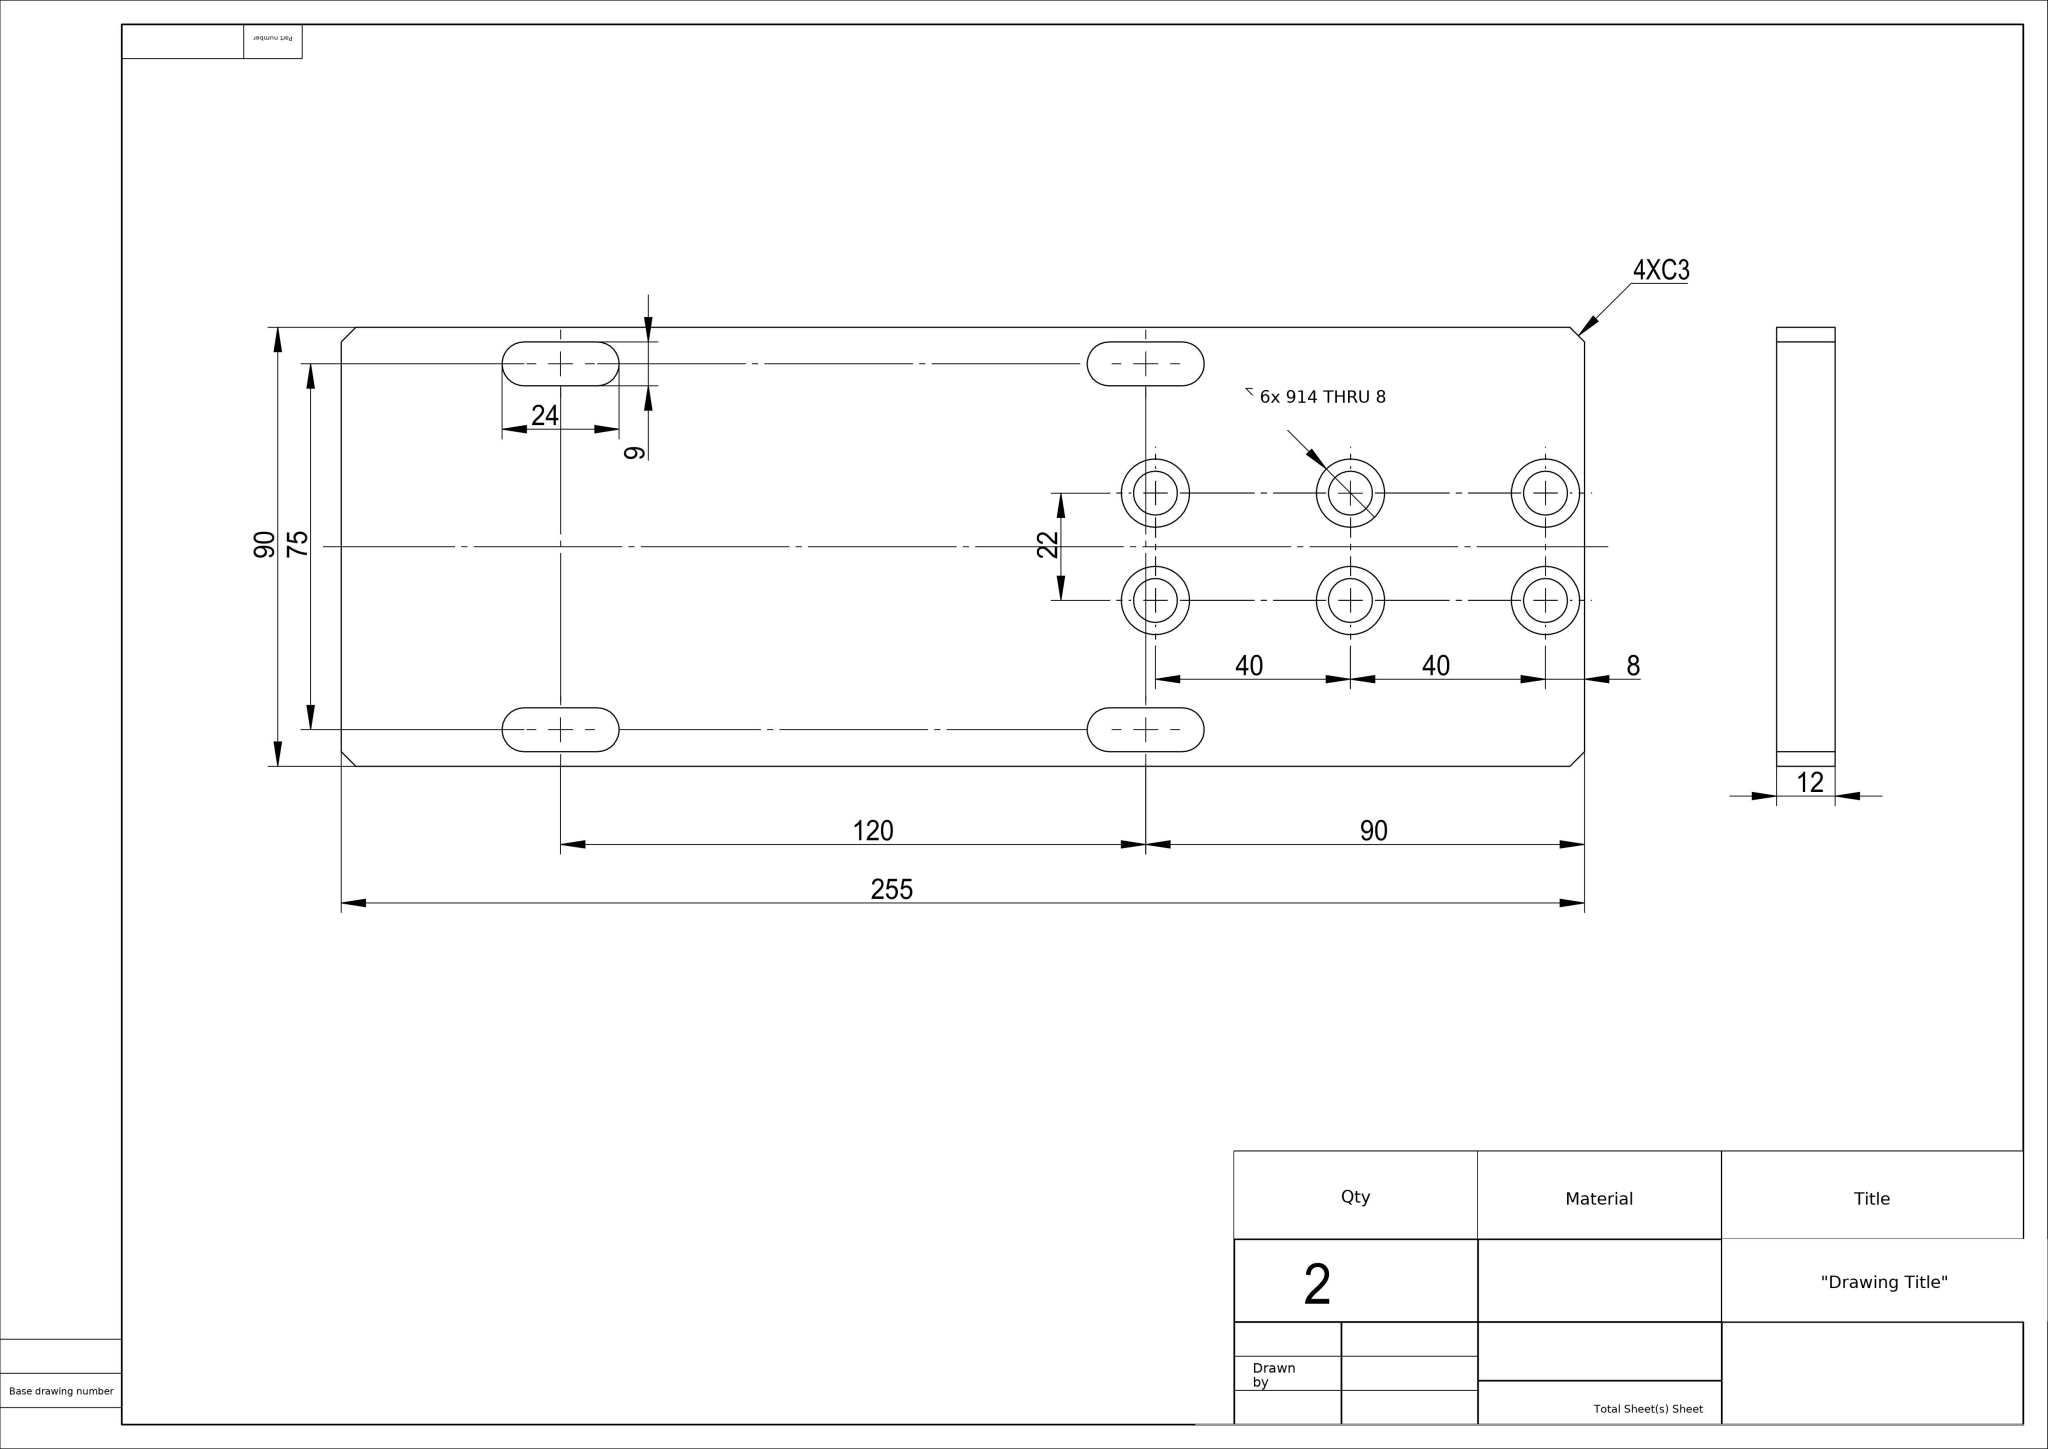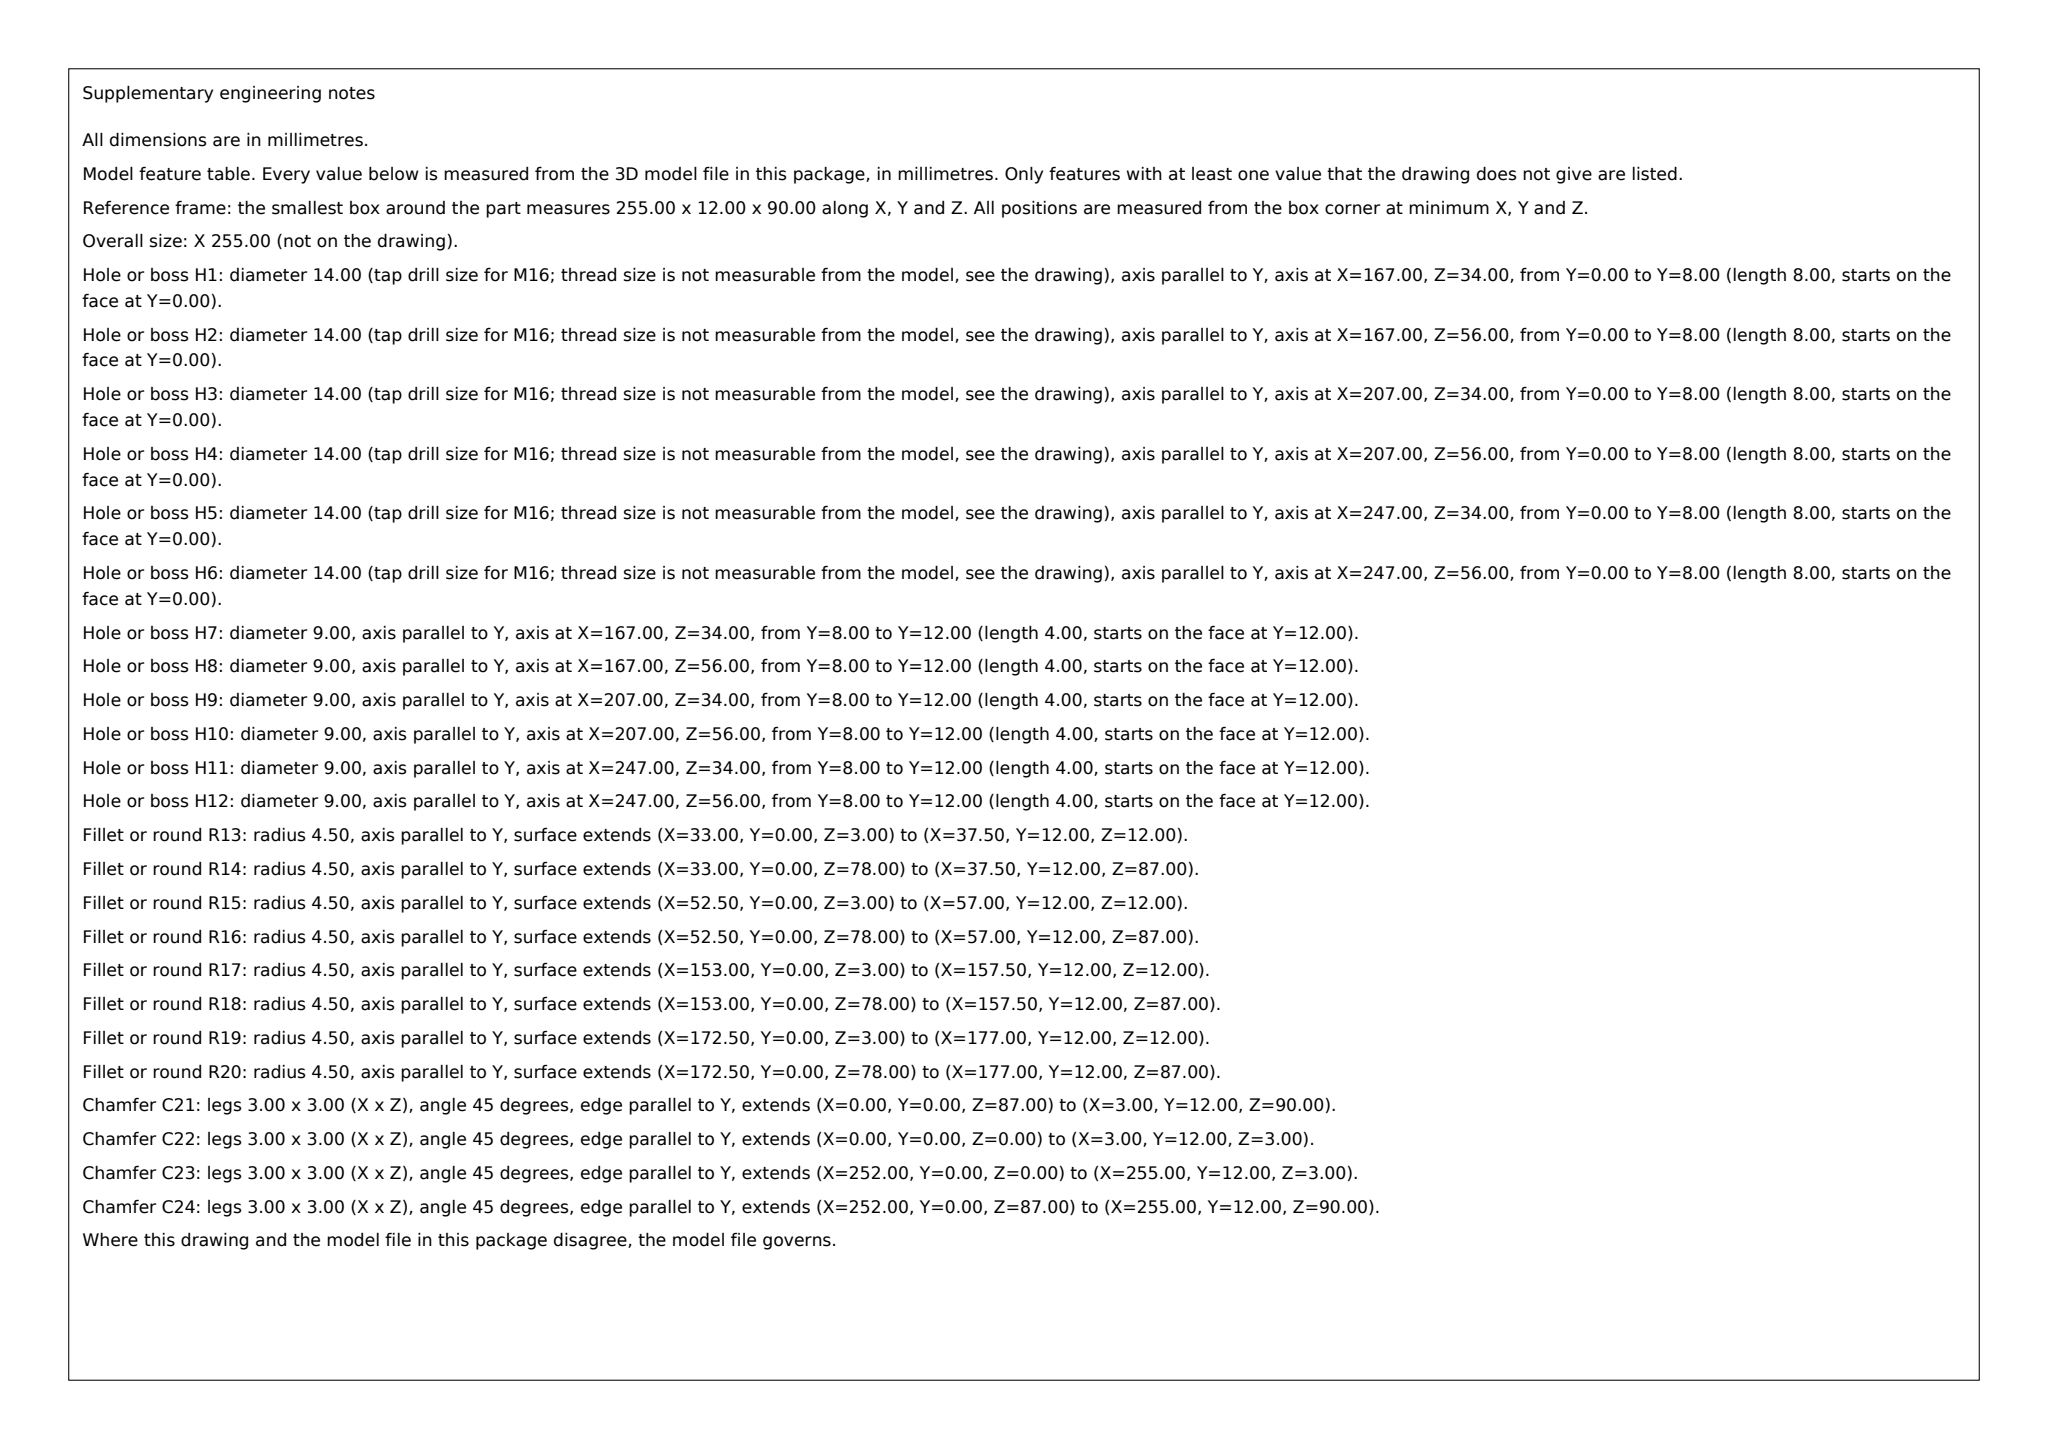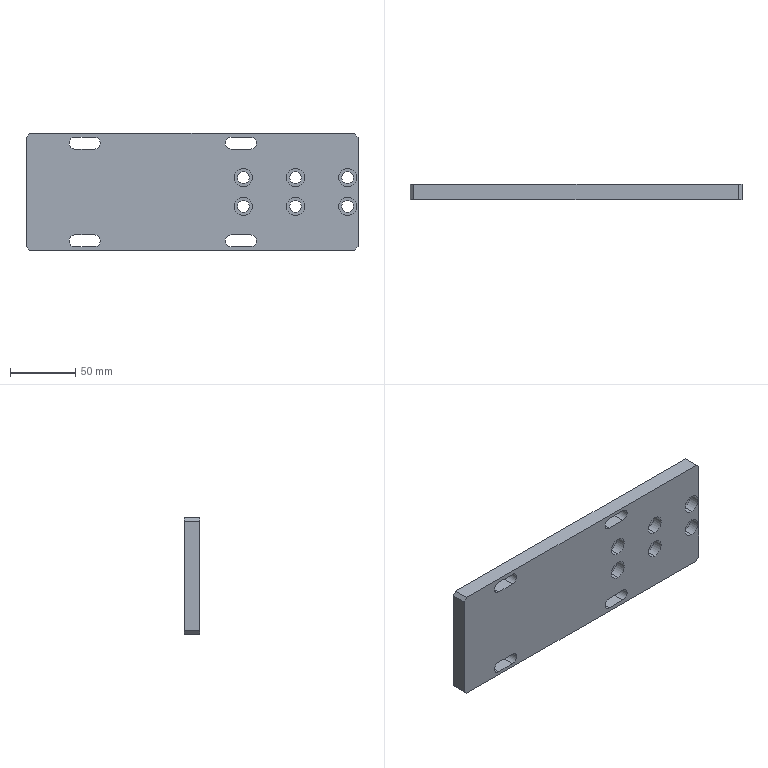Part | SolidWorks | mm | 1 solid | 56 faces | box 255 x 12 x 90 mm | volume 256735 mm3 | cylinder 32 | plane 24 | commonest cylinder face diameters 9 x20 14 x12
build123d program:
from build123d import *

# Parameters (mm, degrees)
SKETCH1_W                                            = 255
SKETCH1_H                                            = 90
BOSS_EXTRUDE1_DEPTH                                  = 12
CUT_EXTRUDE1_DEPTH                                   = 136.74
M8_HEX_HEAD_BOLT_CYLINDRICAL_COUNTERSINK_D           = 9
M8_HEX_HEAD_BOLT_CYLINDRICAL_COUNTERSINK_CBORE_D     = 14
M8_HEX_HEAD_BOLT_CYLINDRICAL_COUNTERSINK_CBORE_DEPTH = 8
LPATTERN1_COUNT                                      = 3
LPATTERN1_PITCH                                      = 40
LPATTERN1_COUNT_DIR2                                 = 2
LPATTERN1_PITCH_DIR2                                 = 22
CHAMFER1_SIZE                                        = 3


with BuildPart() as part:
    # Sketch1 → Boss-Extrude1 (new body)
    with BuildSketch(Plane(origin=(0, 0, 0), x_dir=(1, 0, 0), z_dir=(0, 1, 0))):
        Rectangle(SKETCH1_W, SKETCH1_H)
    extrude(amount=BOSS_EXTRUDE1_DEPTH)

    # Sketch2 → Cut-Extrude1 (cut, through all)
    with BuildSketch(Plane(origin=(0, 12, 0), x_dir=(1, 0, 0), z_dir=(0, 1, 0))):
        with BuildLine():
            Line((-90, 42), (-75, 42))
            ThreePointArc((-75, 42), (-70.5, 37.5), (-75, 33))
            Line((-75, 33), (-90, 33))
            ThreePointArc((-90, 33), (-94.5, 37.5), (-90, 42))
        make_face()
        with BuildLine():
            Line((30, 42), (45, 42))
            ThreePointArc((45, 42), (49.5, 37.5), (45, 33))
            Line((45, 33), (30, 33))
            ThreePointArc((30, 33), (25.5, 37.5), (30, 42))
        make_face()
        with BuildLine():
            Line((-90, -33), (-75, -33))
            ThreePointArc((-75, -33), (-70.5, -37.5), (-75, -42))
            Line((-75, -42), (-90, -42))
            ThreePointArc((-90, -42), (-94.5, -37.5), (-90, -33))
        make_face()
        with BuildLine():
            Line((30, -33), (45, -33))
            ThreePointArc((45, -33), (49.5, -37.5), (45, -42))
            Line((45, -42), (30, -42))
            ThreePointArc((30, -42), (25.5, -37.5), (30, -33))
        make_face()
    extrude(amount=-CUT_EXTRUDE1_DEPTH, mode=Mode.SUBTRACT)

    # M8 Hex Head Bolt Cylindrical Countersink (through all)
    with Locations(Plane(origin=(0, 0, 0), x_dir=(-1, 0, 0), z_dir=(0, -1, 0))):
        with Locations((-119.5, -11)):
            m8_hex_head_bolt_cylindrical_countersink = CounterBoreHole(M8_HEX_HEAD_BOLT_CYLINDRICAL_COUNTERSINK_D / 2, M8_HEX_HEAD_BOLT_CYLINDRICAL_COUNTERSINK_CBORE_D / 2, M8_HEX_HEAD_BOLT_CYLINDRICAL_COUNTERSINK_CBORE_DEPTH)

    # LPattern1: M8 Hex Head Bolt Cylindrical Countersink 3 × 2
    with Locations(*[(-i * LPATTERN1_PITCH, 0, -j * LPATTERN1_PITCH_DIR2) for i in range(LPATTERN1_COUNT) for j in range(LPATTERN1_COUNT_DIR2) if (i, j) != (0, 0)]):
        add(m8_hex_head_bolt_cylindrical_countersink, mode=Mode.SUBTRACT)

    # Chamfer1
    chamfer1_edges = [part.edges().sort_by_distance(p)[0] for p in [
        (127.5, 6, 45),
        (-127.5, 6, 45),
        (-127.5, 6, -45),
        (127.5, 6, -45),
    ]]
    chamfer(chamfer1_edges, length=CHAMFER1_SIZE)


solid = part.part